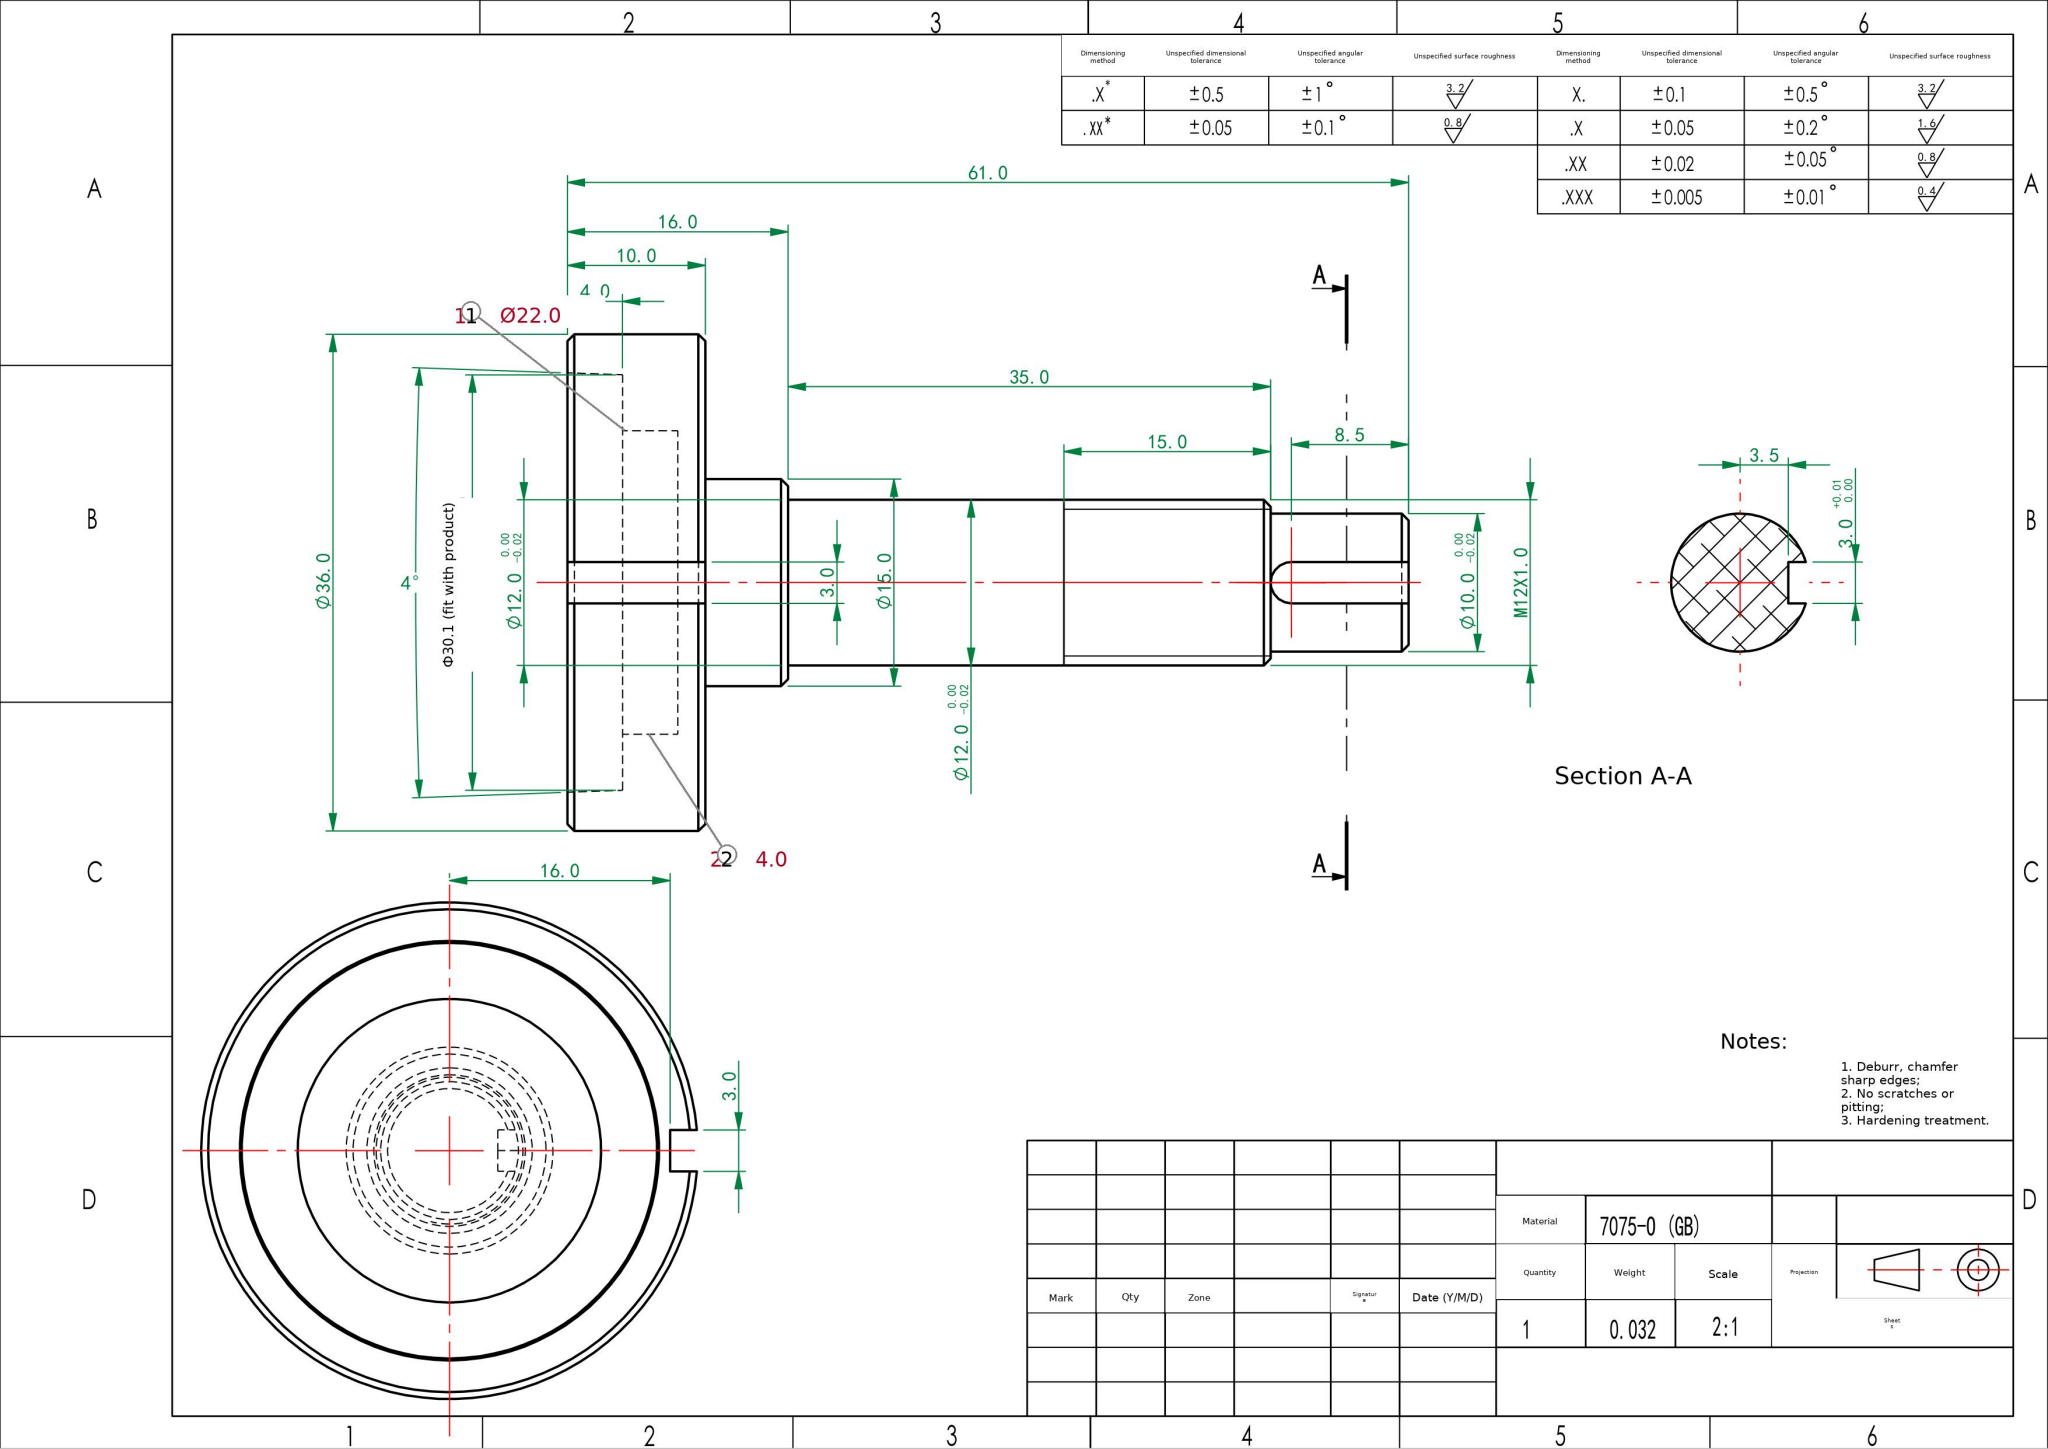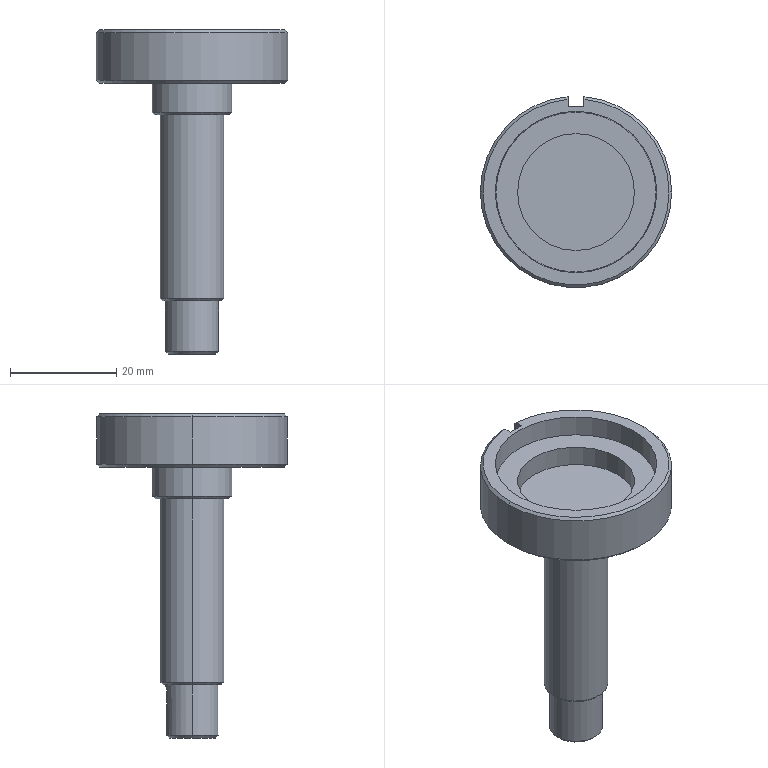Part | SolidWorks | mm | material 7075-0 (GB) | 1 solid | 42 faces | box 36 x 35.94 x 61 mm | volume 11444 mm3 | cone 15 | cylinder 14 | plane 13 | commonest cylinder face diameters 10 x3 36 x3 22 x2 12 x2 15 x2 3 x2